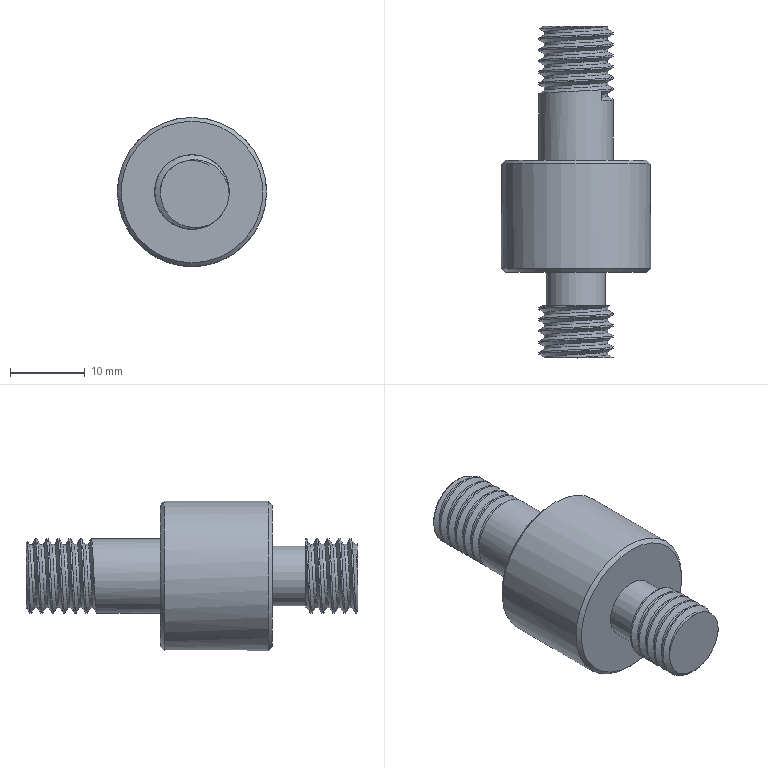Component | NX | MODEL2 | 2 solids | 25 faces | volume 6684 mm3 | cylinder 11 | plane 7 | spline 4 | cone 3 | commonest cylinder face diameters 10 x7 8.5 x2 20 x1 8 x1